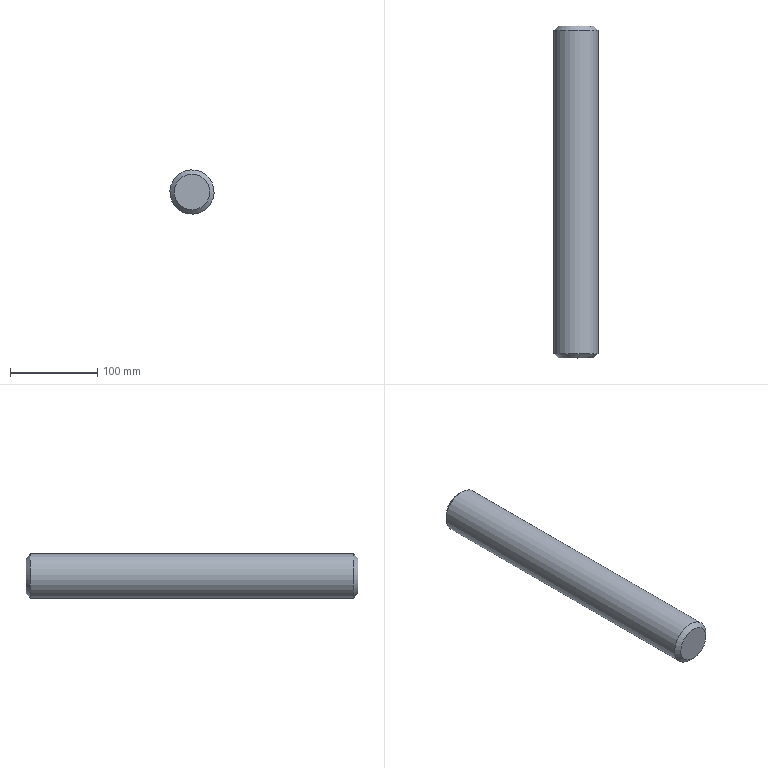Component | NX | PIN_381 | 1 solid | 5 faces | volume 768494 mm3 | plane 2 | cone 2 | cylinder 1 | commonest cylinder face diameters 50.8 x1